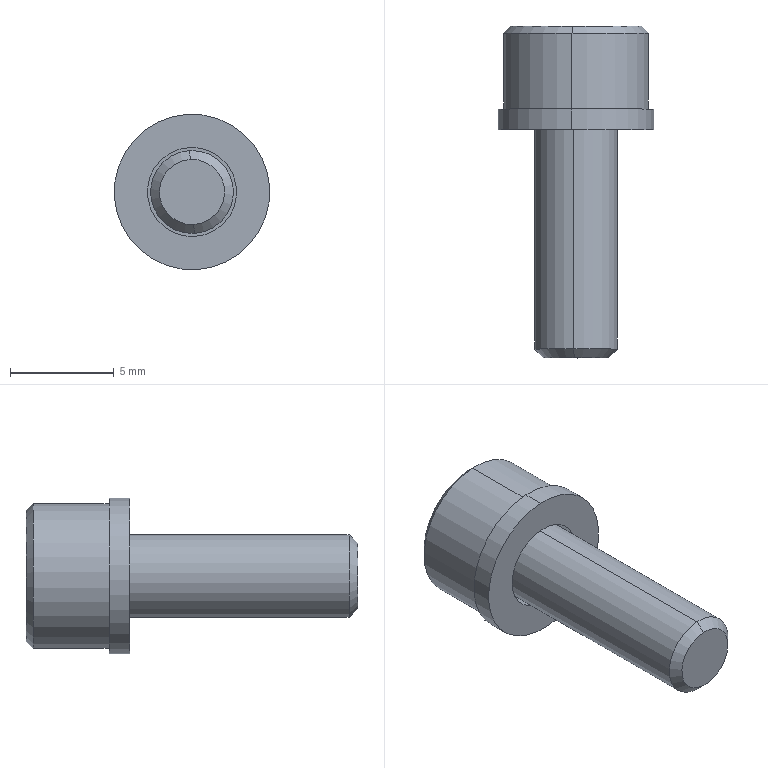Component | SolidWorks | TAC01-M4-L12-2 | 2 solids | 31 faces | box 7.5 x 16 x 7.5 mm | volume 314 mm3 | plane 17 | cylinder 8 | cone 6 | commonest cylinder face diameters 4.3 x2 7.5 x2 4 x2 7 x2
STEP:
#1=COLOUR_RGB('',0.7922,0.8196,0.9333);
#2=FILL_AREA_STYLE_COLOUR('',#1);
#3=FILL_AREA_STYLE('',(#2));
#4=SURFACE_STYLE_FILL_AREA(#3);
#5=SURFACE_SIDE_STYLE('',(#4));
#6=SURFACE_STYLE_USAGE(.BOTH.,#5);
#7=PRESENTATION_STYLE_ASSIGNMENT((#6));
#8=CARTESIAN_POINT('',(9.788,-21.078,0.1048));
#9=VERTEX_POINT('',#8);
#10=CARTESIAN_POINT('',(9.779,-21.078,0.2621));
#11=VERTEX_POINT('',#10);
#12=CARTESIAN_POINT('',(9.783,-21.078,0.1834));
#13=DIRECTION('',(0.,1.,-0.));
#14=DIRECTION('',(0.05512,0.,-0.9985));
#15=AXIS2_PLACEMENT_3D('',#12,#13,#14);
#16=CIRCLE('',#15,0.07874);
#17=EDGE_CURVE('',#9,#11,#16,.T.);
#18=ORIENTED_EDGE('',*,*,#17,.T.);
#19=CARTESIAN_POINT('',(9.779,-20.622,0.2621));
#20=VERTEX_POINT('',#19);
#21=CARTESIAN_POINT('',(9.779,-21.095,0.2621));
#22=DIRECTION('',(0.,1.,-0.));
#23=VECTOR('',#22,39.37);
#24=LINE('',#21,#23);
#25=EDGE_CURVE('',#11,#20,#24,.T.);
#26=ORIENTED_EDGE('',*,*,#25,.T.);
#27=CARTESIAN_POINT('',(9.788,-20.622,0.1048));
#28=VERTEX_POINT('',#27);
#29=CARTESIAN_POINT('',(9.783,-20.622,0.1834));
#30=DIRECTION('',(-0.,-1.,0.));
#31=DIRECTION('',(0.05512,0.,-0.9985));
#32=AXIS2_PLACEMENT_3D('',#29,#30,#31);
#33=CIRCLE('',#32,0.07874);
#34=EDGE_CURVE('',#20,#28,#33,.T.);
#35=ORIENTED_EDGE('',*,*,#34,.T.);
#36=CARTESIAN_POINT('',(9.788,-21.095,0.1048));
#37=DIRECTION('',(0.,1.,-0.));
#38=VECTOR('',#37,39.37);
#39=LINE('',#36,#38);
#40=EDGE_CURVE('',#9,#28,#39,.T.);
#41=ORIENTED_EDGE('',*,*,#40,.F.);
#42=EDGE_LOOP('',(#18,#26,#35,#41));
#43=FACE_OUTER_BOUND('',#42,.T.);
#44=CARTESIAN_POINT('',(9.783,-21.095,0.1834));
#45=DIRECTION('',(0.,1.,-0.));
#46=DIRECTION('',(0.05512,0.,-0.9985));
#47=AXIS2_PLACEMENT_3D('',#44,#45,#46);
#48=CYLINDRICAL_SURFACE('',#47,0.07874);
#49=ADVANCED_FACE('',(#43),#48,.T.);
#50=CARTESIAN_POINT('',(9.787,-21.095,0.1217));
#51=VERTEX_POINT('',#50);
#52=CARTESIAN_POINT('',(9.78,-21.095,0.2452));
#53=VERTEX_POINT('',#52);
#54=CARTESIAN_POINT('',(9.783,-21.095,0.1834));
#55=DIRECTION('',(0.,1.,-0.));
#56=DIRECTION('',(0.05512,0.,-0.9985));
#57=AXIS2_PLACEMENT_3D('',#54,#55,#56);
#58=CIRCLE('',#57,0.06183);
#59=EDGE_CURVE('',#51,#53,#58,.T.);
#60=ORIENTED_EDGE('',*,*,#59,.T.);
#61=CARTESIAN_POINT('',(9.779,-21.078,0.2621));
#62=DIRECTION('',(-0.03898,0.7071,0.706));
#63=VECTOR('',#62,39.37);
#64=LINE('',#61,#63);
#65=EDGE_CURVE('',#53,#11,#64,.T.);
#66=ORIENTED_EDGE('',*,*,#65,.T.);
#67=ORIENTED_EDGE('',*,*,#17,.F.);
#68=CARTESIAN_POINT('',(9.788,-21.078,0.1048));
#69=DIRECTION('',(0.03898,0.7071,-0.706));
#70=VECTOR('',#69,39.37);
#71=LINE('',#68,#70);
#72=EDGE_CURVE('',#51,#9,#71,.T.);
#73=ORIENTED_EDGE('',*,*,#72,.F.);
#74=EDGE_LOOP('',(#60,#66,#67,#73));
#75=FACE_OUTER_BOUND('',#74,.T.);
#76=CARTESIAN_POINT('',(9.783,-21.078,0.1834));
#77=DIRECTION('',(0.,1.,-0.));
#78=DIRECTION('',(0.05512,0.,-0.9985));
#79=AXIS2_PLACEMENT_3D('',#76,#77,#78);
#80=CONICAL_SURFACE('',#79,0.07874,0.7854);
#81=ADVANCED_FACE('',(#75),#80,.T.);
#82=CARTESIAN_POINT('',(9.791,-20.622,0.04586));
#83=VERTEX_POINT('',#82);
#84=CARTESIAN_POINT('',(9.776,-20.622,0.321));
#85=VERTEX_POINT('',#84);
#86=CARTESIAN_POINT('',(9.783,-20.622,0.1834));
#87=DIRECTION('',(0.,1.,-0.));
#88=DIRECTION('',(0.05512,0.,-0.9985));
#89=AXIS2_PLACEMENT_3D('',#86,#87,#88);
#90=CIRCLE('',#89,0.1378);
#91=EDGE_CURVE('',#83,#85,#90,.T.);
#92=ORIENTED_EDGE('',*,*,#91,.T.);
#93=CARTESIAN_POINT('',(9.776,-20.479,0.321));
#94=VERTEX_POINT('',#93);
#95=CARTESIAN_POINT('',(9.776,-20.622,0.321));
#96=DIRECTION('',(0.,1.,-0.));
#97=VECTOR('',#96,39.37);
#98=LINE('',#95,#97);
#99=EDGE_CURVE('',#85,#94,#98,.T.);
#100=ORIENTED_EDGE('',*,*,#99,.T.);
#101=CARTESIAN_POINT('',(9.791,-20.479,0.04586));
#102=VERTEX_POINT('',#101);
#103=CARTESIAN_POINT('',(9.783,-20.479,0.1834));
#104=DIRECTION('',(-0.,-1.,0.));
#105=DIRECTION('',(0.05512,0.,-0.9985));
#106=AXIS2_PLACEMENT_3D('',#103,#104,#105);
#107=CIRCLE('',#106,0.1378);
#108=EDGE_CURVE('',#94,#102,#107,.T.);
#109=ORIENTED_EDGE('',*,*,#108,.T.);
#110=CARTESIAN_POINT('',(9.791,-20.622,0.04586));
#111=DIRECTION('',(0.,1.,-0.));
#112=VECTOR('',#111,39.37);
#113=LINE('',#110,#112);
#114=EDGE_CURVE('',#83,#102,#113,.T.);
#115=ORIENTED_EDGE('',*,*,#114,.F.);
#116=EDGE_LOOP('',(#92,#100,#109,#115));
#117=FACE_OUTER_BOUND('',#116,.T.);
#118=CARTESIAN_POINT('',(9.783,-20.622,0.1834));
#119=DIRECTION('',(0.,1.,-0.));
#120=DIRECTION('',(0.05512,0.,-0.9985));
#121=AXIS2_PLACEMENT_3D('',#118,#119,#120);
#122=CYLINDRICAL_SURFACE('',#121,0.1378);
#123=ADVANCED_FACE('',(#117),#122,.T.);
#124=CARTESIAN_POINT('',(9.777,-20.465,0.3073));
#125=VERTEX_POINT('',#124);
#126=CARTESIAN_POINT('',(9.79,-20.465,0.05962));
#127=VERTEX_POINT('',#126);
#128=CARTESIAN_POINT('',(9.783,-20.465,0.1834));
#129=DIRECTION('',(-0.,-1.,0.));
#130=DIRECTION('',(-0.05512,0.,0.9985));
#131=AXIS2_PLACEMENT_3D('',#128,#129,#130);
#132=CIRCLE('',#131,0.124);
#133=EDGE_CURVE('',#125,#127,#132,.T.);
#134=ORIENTED_EDGE('',*,*,#133,.T.);
#135=CARTESIAN_POINT('',(9.791,-20.479,0.04586));
#136=DIRECTION('',(0.03898,-0.7071,-0.706));
#137=VECTOR('',#136,39.37);
#138=LINE('',#135,#137);
#139=EDGE_CURVE('',#127,#102,#138,.T.);
#140=ORIENTED_EDGE('',*,*,#139,.T.);
#141=ORIENTED_EDGE('',*,*,#108,.F.);
#142=CARTESIAN_POINT('',(9.776,-20.479,0.321));
#143=DIRECTION('',(-0.03898,-0.7071,0.706));
#144=VECTOR('',#143,39.37);
#145=LINE('',#142,#144);
#146=EDGE_CURVE('',#125,#94,#145,.T.);
#147=ORIENTED_EDGE('',*,*,#146,.F.);
#148=EDGE_LOOP('',(#134,#140,#141,#147));
#149=FACE_OUTER_BOUND('',#148,.T.);
#150=CARTESIAN_POINT('',(9.783,-20.479,0.1834));
#151=DIRECTION('',(-0.,-1.,0.));
#152=DIRECTION('',(-0.05512,0.,0.9985));
#153=AXIS2_PLACEMENT_3D('',#150,#151,#152);
#154=CONICAL_SURFACE('',#153,0.1378,0.7854);
#155=ADVANCED_FACE('',(#149),#154,.T.);
#156=CARTESIAN_POINT('',(9.783,-20.578,0.1834));
#157=VERTEX_POINT('',#156);
#158=CARTESIAN_POINT('',(9.842,-20.544,0.1867));
#159=VERTEX_POINT('',#158);
#160=CARTESIAN_POINT('',(9.842,-20.544,0.1867));
#161=DIRECTION('',(0.8647,0.5,0.04774));
#162=VECTOR('',#161,39.37);
#163=LINE('',#160,#162);
#164=EDGE_CURVE('',#157,#159,#163,.T.);
#165=ORIENTED_EDGE('',*,*,#164,.F.);
#166=CARTESIAN_POINT('',(9.724,-20.544,0.1802));
#167=VERTEX_POINT('',#166);
#168=CARTESIAN_POINT('',(9.724,-20.544,0.1802));
#169=DIRECTION('',(-0.8647,0.5,-0.04774));
#170=VECTOR('',#169,39.37);
#171=LINE('',#168,#170);
#172=EDGE_CURVE('',#157,#167,#171,.T.);
#173=ORIENTED_EDGE('',*,*,#172,.T.);
#174=CARTESIAN_POINT('',(9.731,-20.544,0.2101));
#175=VERTEX_POINT('',#174);
#176=CARTESIAN_POINT('',(9.783,-20.544,0.1834));
#177=DIRECTION('',(-0.,-1.,0.));
#178=DIRECTION('',(0.9985,0.,0.05512));
#179=AXIS2_PLACEMENT_3D('',#176,#177,#178);
#180=CIRCLE('',#179,0.05906);
#181=EDGE_CURVE('',#175,#167,#180,.T.);
#182=ORIENTED_EDGE('',*,*,#181,.F.);
#183=CARTESIAN_POINT('',(9.78,-20.544,0.2424));
#184=VERTEX_POINT('',#183);
#185=CARTESIAN_POINT('',(9.783,-20.544,0.1834));
#186=DIRECTION('',(-0.,-1.,0.));
#187=DIRECTION('',(0.9985,0.,0.05512));
#188=AXIS2_PLACEMENT_3D('',#185,#186,#187);
#189=CIRCLE('',#188,0.05906);
#190=EDGE_CURVE('',#184,#175,#189,.T.);
#191=ORIENTED_EDGE('',*,*,#190,.F.);
#192=CARTESIAN_POINT('',(9.833,-20.544,0.2157));
#193=VERTEX_POINT('',#192);
#194=CARTESIAN_POINT('',(9.783,-20.544,0.1834));
#195=DIRECTION('',(-0.,-1.,0.));
#196=DIRECTION('',(0.9985,0.,0.05512));
#197=AXIS2_PLACEMENT_3D('',#194,#195,#196);
#198=CIRCLE('',#197,0.05906);
#199=EDGE_CURVE('',#193,#184,#198,.T.);
#200=ORIENTED_EDGE('',*,*,#199,.F.);
#201=CARTESIAN_POINT('',(9.783,-20.544,0.1834));
#202=DIRECTION('',(-0.,-1.,0.));
#203=DIRECTION('',(0.9985,0.,0.05512));
#204=AXIS2_PLACEMENT_3D('',#201,#202,#203);
#205=CIRCLE('',#204,0.05906);
#206=EDGE_CURVE('',#159,#193,#205,.T.);
#207=ORIENTED_EDGE('',*,*,#206,.F.);
#208=EDGE_LOOP('',(#165,#173,#182,#191,#200,#207));
#209=FACE_OUTER_BOUND('',#208,.T.);
#210=CARTESIAN_POINT('',(9.783,-20.544,0.1834));
#211=DIRECTION('',(0.,1.,-0.));
#212=DIRECTION('',(0.9985,0.,0.05512));
#213=AXIS2_PLACEMENT_3D('',#210,#211,#212);
#214=CONICAL_SURFACE('',#213,0.05906,1.047);
#215=ADVANCED_FACE('',(#209),#214,.F.);
#216=ORIENTED_EDGE('',*,*,#25,.F.);
#217=CARTESIAN_POINT('',(9.783,-21.078,0.1834));
#218=DIRECTION('',(0.,1.,-0.));
#219=DIRECTION('',(0.05512,0.,-0.9985));
#220=AXIS2_PLACEMENT_3D('',#217,#218,#219);
#221=CIRCLE('',#220,0.07874);
#222=EDGE_CURVE('',#11,#9,#221,.T.);
#223=ORIENTED_EDGE('',*,*,#222,.T.);
#224=ORIENTED_EDGE('',*,*,#40,.T.);
#225=CARTESIAN_POINT('',(9.783,-20.622,0.1834));
#226=DIRECTION('',(-0.,-1.,0.));
#227=DIRECTION('',(0.05512,0.,-0.9985));
#228=AXIS2_PLACEMENT_3D('',#225,#226,#227);
#229=CIRCLE('',#228,0.07874);
#230=EDGE_CURVE('',#28,#20,#229,.T.);
#231=ORIENTED_EDGE('',*,*,#230,.T.);
#232=EDGE_LOOP('',(#216,#223,#224,#231));
#233=FACE_OUTER_BOUND('',#232,.T.);
#234=CARTESIAN_POINT('',(9.783,-21.095,0.1834));
#235=DIRECTION('',(0.,1.,-0.));
#236=DIRECTION('',(0.05512,0.,-0.9985));
#237=AXIS2_PLACEMENT_3D('',#234,#235,#236);
#238=CYLINDRICAL_SURFACE('',#237,0.07874);
#239=ADVANCED_FACE('',(#233),#238,.T.);
#240=ORIENTED_EDGE('',*,*,#91,.F.);
#241=CARTESIAN_POINT('',(9.783,-20.622,0.1834));
#242=DIRECTION('',(0.,1.,-0.));
#243=DIRECTION('',(0.05512,0.,-0.9985));
#244=AXIS2_PLACEMENT_3D('',#241,#242,#243);
#245=CIRCLE('',#244,0.1378);
#246=EDGE_CURVE('',#85,#83,#245,.T.);
#247=ORIENTED_EDGE('',*,*,#246,.F.);
#248=EDGE_LOOP('',(#240,#247));
#249=FACE_OUTER_BOUND('',#248,.T.);
#250=ORIENTED_EDGE('',*,*,#230,.F.);
#251=ORIENTED_EDGE('',*,*,#34,.F.);
#252=EDGE_LOOP('',(#250,#251));
#253=FACE_BOUND('',#252,.T.);
#254=CARTESIAN_POINT('',(9.646,-20.622,0.1759));
#255=DIRECTION('',(0.,1.,-0.));
#256=DIRECTION('',(0.05512,-0.,-0.9985));
#257=AXIS2_PLACEMENT_3D('',#254,#255,#256);
#258=PLANE('',#257);
#259=ADVANCED_FACE('',(#249,#253),#258,.F.);
#260=ORIENTED_EDGE('',*,*,#65,.F.);
#261=CARTESIAN_POINT('',(9.783,-21.095,0.1834));
#262=DIRECTION('',(0.,1.,-0.));
#263=DIRECTION('',(0.05512,0.,-0.9985));
#264=AXIS2_PLACEMENT_3D('',#261,#262,#263);
#265=CIRCLE('',#264,0.06183);
#266=EDGE_CURVE('',#53,#51,#265,.T.);
#267=ORIENTED_EDGE('',*,*,#266,.T.);
#268=ORIENTED_EDGE('',*,*,#72,.T.);
#269=ORIENTED_EDGE('',*,*,#222,.F.);
#270=EDGE_LOOP('',(#260,#267,#268,#269));
#271=FACE_OUTER_BOUND('',#270,.T.);
#272=CARTESIAN_POINT('',(9.783,-21.078,0.1834));
#273=DIRECTION('',(0.,1.,-0.));
#274=DIRECTION('',(0.05512,0.,-0.9985));
#275=AXIS2_PLACEMENT_3D('',#272,#273,#274);
#276=CONICAL_SURFACE('',#275,0.07874,0.7854);
#277=ADVANCED_FACE('',(#271),#276,.T.);
#278=ORIENTED_EDGE('',*,*,#99,.F.);
#279=ORIENTED_EDGE('',*,*,#246,.T.);
#280=ORIENTED_EDGE('',*,*,#114,.T.);
#281=CARTESIAN_POINT('',(9.783,-20.479,0.1834));
#282=DIRECTION('',(-0.,-1.,0.));
#283=DIRECTION('',(0.05512,0.,-0.9985));
#284=AXIS2_PLACEMENT_3D('',#281,#282,#283);
#285=CIRCLE('',#284,0.1378);
#286=EDGE_CURVE('',#102,#94,#285,.T.);
#287=ORIENTED_EDGE('',*,*,#286,.T.);
#288=EDGE_LOOP('',(#278,#279,#280,#287));
#289=FACE_OUTER_BOUND('',#288,.T.);
#290=CARTESIAN_POINT('',(9.783,-20.622,0.1834));
#291=DIRECTION('',(0.,1.,-0.));
#292=DIRECTION('',(0.05512,0.,-0.9985));
#293=AXIS2_PLACEMENT_3D('',#290,#291,#292);
#294=CYLINDRICAL_SURFACE('',#293,0.1378);
#295=ADVANCED_FACE('',(#289),#294,.T.);
#296=ORIENTED_EDGE('',*,*,#59,.F.);
#297=ORIENTED_EDGE('',*,*,#266,.F.);
#298=EDGE_LOOP('',(#296,#297));
#299=FACE_OUTER_BOUND('',#298,.T.);
#300=CARTESIAN_POINT('',(9.722,-21.095,0.18));
#301=DIRECTION('',(0.,1.,-0.));
#302=DIRECTION('',(0.05512,-0.,-0.9985));
#303=AXIS2_PLACEMENT_3D('',#300,#301,#302);
#304=PLANE('',#303);
#305=ADVANCED_FACE('',(#299),#304,.F.);
#306=ORIENTED_EDGE('',*,*,#139,.F.);
#307=CARTESIAN_POINT('',(9.783,-20.465,0.1834));
#308=DIRECTION('',(-0.,-1.,0.));
#309=DIRECTION('',(-0.05512,0.,0.9985));
#310=AXIS2_PLACEMENT_3D('',#307,#308,#309);
#311=CIRCLE('',#310,0.124);
#312=EDGE_CURVE('',#127,#125,#311,.T.);
#313=ORIENTED_EDGE('',*,*,#312,.T.);
#314=ORIENTED_EDGE('',*,*,#146,.T.);
#315=ORIENTED_EDGE('',*,*,#286,.F.);
#316=EDGE_LOOP('',(#306,#313,#314,#315));
#317=FACE_OUTER_BOUND('',#316,.T.);
#318=CARTESIAN_POINT('',(9.783,-20.479,0.1834));
#319=DIRECTION('',(-0.,-1.,0.));
#320=DIRECTION('',(-0.05512,0.,0.9985));
#321=AXIS2_PLACEMENT_3D('',#318,#319,#320);
#322=CONICAL_SURFACE('',#321,0.1378,0.7854);
#323=ADVANCED_FACE('',(#317),#322,.T.);
#324=CARTESIAN_POINT('',(9.852,-20.465,0.1872));
#325=VERTEX_POINT('',#324);
#326=CARTESIAN_POINT('',(9.814,-20.465,0.2443));
#327=VERTEX_POINT('',#326);
#328=CARTESIAN_POINT('',(9.814,-20.465,0.2443));
#329=DIRECTION('',(-0.547,0.,0.8371));
#330=VECTOR('',#329,39.37);
#331=LINE('',#328,#330);
#332=EDGE_CURVE('',#325,#327,#331,.T.);
#333=ORIENTED_EDGE('',*,*,#332,.T.);
#334=CARTESIAN_POINT('',(9.746,-20.465,0.2405));
#335=VERTEX_POINT('',#334);
#336=CARTESIAN_POINT('',(9.746,-20.465,0.2405));
#337=DIRECTION('',(-0.9985,0.,-0.05512));
#338=VECTOR('',#337,39.37);
#339=LINE('',#336,#338);
#340=EDGE_CURVE('',#327,#335,#339,.T.);
#341=ORIENTED_EDGE('',*,*,#340,.T.);
#342=CARTESIAN_POINT('',(9.715,-20.465,0.1797));
#343=VERTEX_POINT('',#342);
#344=CARTESIAN_POINT('',(9.715,-20.465,0.1797));
#345=DIRECTION('',(-0.4515,0.,-0.8923));
#346=VECTOR('',#345,39.37);
#347=LINE('',#344,#346);
#348=EDGE_CURVE('',#335,#343,#347,.T.);
#349=ORIENTED_EDGE('',*,*,#348,.T.);
#350=CARTESIAN_POINT('',(9.753,-20.465,0.1226));
#351=VERTEX_POINT('',#350);
#352=CARTESIAN_POINT('',(9.753,-20.465,0.1226));
#353=DIRECTION('',(0.547,-0.,-0.8371));
#354=VECTOR('',#353,39.37);
#355=LINE('',#352,#354);
#356=EDGE_CURVE('',#343,#351,#355,.T.);
#357=ORIENTED_EDGE('',*,*,#356,.T.);
#358=CARTESIAN_POINT('',(9.821,-20.465,0.1264));
#359=VERTEX_POINT('',#358);
#360=CARTESIAN_POINT('',(9.821,-20.465,0.1264));
#361=DIRECTION('',(0.9985,-0.,0.05512));
#362=VECTOR('',#361,39.37);
#363=LINE('',#360,#362);
#364=EDGE_CURVE('',#351,#359,#363,.T.);
#365=ORIENTED_EDGE('',*,*,#364,.T.);
#366=CARTESIAN_POINT('',(9.852,-20.465,0.1872));
#367=DIRECTION('',(-0.4515,0.,-0.8923));
#368=VECTOR('',#367,39.37);
#369=LINE('',#366,#368);
#370=EDGE_CURVE('',#325,#359,#369,.T.);
#371=ORIENTED_EDGE('',*,*,#370,.F.);
#372=EDGE_LOOP('',(#333,#341,#349,#357,#365,#371));
#373=FACE_BOUND('',#372,.T.);
#374=ORIENTED_EDGE('',*,*,#133,.F.);
#375=ORIENTED_EDGE('',*,*,#312,.F.);
#376=EDGE_LOOP('',(#374,#375));
#377=FACE_OUTER_BOUND('',#376,.T.);
#378=CARTESIAN_POINT('',(9.783,-20.465,0.1834));
#379=DIRECTION('',(-0.,-1.,0.));
#380=DIRECTION('',(-0.05512,0.,0.9985));
#381=AXIS2_PLACEMENT_3D('',#378,#379,#380);
#382=PLANE('',#381);
#383=ADVANCED_FACE('',(#373,#377),#382,.F.);
#384=CARTESIAN_POINT('',(9.821,-20.544,0.1264));
#385=VERTEX_POINT('',#384);
#386=CARTESIAN_POINT('',(9.821,-20.544,0.1264));
#387=DIRECTION('',(0.,1.,-0.));
#388=VECTOR('',#387,39.37);
#389=LINE('',#386,#388);
#390=EDGE_CURVE('',#385,#359,#389,.T.);
#391=ORIENTED_EDGE('',*,*,#390,.F.);
#392=CARTESIAN_POINT('',(9.836,-20.544,0.1568));
#393=VERTEX_POINT('',#392);
#394=CARTESIAN_POINT('',(9.852,-20.544,0.1872));
#395=DIRECTION('',(-0.4515,0.,-0.8923));
#396=VECTOR('',#395,39.37);
#397=LINE('',#394,#396);
#398=EDGE_CURVE('',#393,#385,#397,.T.);
#399=ORIENTED_EDGE('',*,*,#398,.F.);
#400=CARTESIAN_POINT('',(9.852,-20.544,0.1872));
#401=VERTEX_POINT('',#400);
#402=CARTESIAN_POINT('',(9.852,-20.544,0.1872));
#403=DIRECTION('',(-0.4515,0.,-0.8923));
#404=VECTOR('',#403,39.37);
#405=LINE('',#402,#404);
#406=EDGE_CURVE('',#401,#393,#405,.T.);
#407=ORIENTED_EDGE('',*,*,#406,.F.);
#408=CARTESIAN_POINT('',(9.852,-20.544,0.1872));
#409=DIRECTION('',(-0.,-1.,0.));
#410=VECTOR('',#409,39.37);
#411=LINE('',#408,#410);
#412=EDGE_CURVE('',#325,#401,#411,.T.);
#413=ORIENTED_EDGE('',*,*,#412,.F.);
#414=ORIENTED_EDGE('',*,*,#370,.T.);
#415=EDGE_LOOP('',(#391,#399,#407,#413,#414));
#416=FACE_OUTER_BOUND('',#415,.T.);
#417=CARTESIAN_POINT('',(9.852,-20.544,0.1872));
#418=DIRECTION('',(0.8923,-0.,-0.4515));
#419=DIRECTION('',(-0.4515,0.,-0.8923));
#420=AXIS2_PLACEMENT_3D('',#417,#418,#419);
#421=PLANE('',#420);
#422=ADVANCED_FACE('',(#416),#421,.F.);
#423=CARTESIAN_POINT('',(9.753,-20.544,0.1226));
#424=VERTEX_POINT('',#423);
#425=CARTESIAN_POINT('',(9.753,-20.544,0.1226));
#426=DIRECTION('',(0.,1.,-0.));
#427=VECTOR('',#426,39.37);
#428=LINE('',#425,#427);
#429=EDGE_CURVE('',#424,#351,#428,.T.);
#430=ORIENTED_EDGE('',*,*,#429,.F.);
#431=CARTESIAN_POINT('',(9.787,-20.544,0.1245));
#432=VERTEX_POINT('',#431);
#433=CARTESIAN_POINT('',(9.821,-20.544,0.1264));
#434=DIRECTION('',(-0.9985,0.,-0.05512));
#435=VECTOR('',#434,39.37);
#436=LINE('',#433,#435);
#437=EDGE_CURVE('',#432,#424,#436,.T.);
#438=ORIENTED_EDGE('',*,*,#437,.F.);
#439=CARTESIAN_POINT('',(9.821,-20.544,0.1264));
#440=DIRECTION('',(-0.9985,0.,-0.05512));
#441=VECTOR('',#440,39.37);
#442=LINE('',#439,#441);
#443=EDGE_CURVE('',#385,#432,#442,.T.);
#444=ORIENTED_EDGE('',*,*,#443,.F.);
#445=ORIENTED_EDGE('',*,*,#390,.T.);
#446=ORIENTED_EDGE('',*,*,#364,.F.);
#447=EDGE_LOOP('',(#430,#438,#444,#445,#446));
#448=FACE_OUTER_BOUND('',#447,.T.);
#449=CARTESIAN_POINT('',(9.821,-20.544,0.1264));
#450=DIRECTION('',(0.05512,-0.,-0.9985));
#451=DIRECTION('',(-0.,-1.,0.));
#452=AXIS2_PLACEMENT_3D('',#449,#450,#451);
#453=PLANE('',#452);
#454=ADVANCED_FACE('',(#448),#453,.F.);
#455=CARTESIAN_POINT('',(9.783,-20.544,0.1834));
#456=DIRECTION('',(-0.,-1.,0.));
#457=DIRECTION('',(0.9985,0.,0.05512));
#458=AXIS2_PLACEMENT_3D('',#455,#456,#457);
#459=CIRCLE('',#458,0.05906);
#460=EDGE_CURVE('',#432,#393,#459,.T.);
#461=ORIENTED_EDGE('',*,*,#460,.T.);
#462=ORIENTED_EDGE('',*,*,#398,.T.);
#463=ORIENTED_EDGE('',*,*,#443,.T.);
#464=EDGE_LOOP('',(#461,#462,#463));
#465=FACE_OUTER_BOUND('',#464,.T.);
#466=CARTESIAN_POINT('',(9.783,-20.544,0.1834));
#467=DIRECTION('',(0.,1.,-0.));
#468=DIRECTION('',(0.05512,-0.,-0.9985));
#469=AXIS2_PLACEMENT_3D('',#466,#467,#468);
#470=PLANE('',#469);
#471=ADVANCED_FACE('',(#465),#470,.T.);
#472=CARTESIAN_POINT('',(9.783,-20.544,0.1834));
#473=DIRECTION('',(-0.,-1.,0.));
#474=DIRECTION('',(0.9985,0.,0.05512));
#475=AXIS2_PLACEMENT_3D('',#472,#473,#474);
#476=CIRCLE('',#475,0.05906);
#477=EDGE_CURVE('',#393,#159,#476,.T.);
#478=ORIENTED_EDGE('',*,*,#477,.T.);
#479=ORIENTED_EDGE('',*,*,#206,.T.);
#480=CARTESIAN_POINT('',(9.833,-20.544,0.2157));
#481=DIRECTION('',(0.547,-0.,-0.8371));
#482=VECTOR('',#481,39.37);
#483=LINE('',#480,#482);
#484=EDGE_CURVE('',#193,#401,#483,.T.);
#485=ORIENTED_EDGE('',*,*,#484,.T.);
#486=ORIENTED_EDGE('',*,*,#406,.T.);
#487=EDGE_LOOP('',(#478,#479,#485,#486));
#488=FACE_OUTER_BOUND('',#487,.T.);
#489=CARTESIAN_POINT('',(9.783,-20.544,0.1834));
#490=DIRECTION('',(0.,1.,-0.));
#491=DIRECTION('',(0.05512,-0.,-0.9985));
#492=AXIS2_PLACEMENT_3D('',#489,#490,#491);
#493=PLANE('',#492);
#494=ADVANCED_FACE('',(#488),#493,.T.);
#495=ORIENTED_EDGE('',*,*,#412,.T.);
#496=ORIENTED_EDGE('',*,*,#484,.F.);
#497=CARTESIAN_POINT('',(9.814,-20.544,0.2443));
#498=VERTEX_POINT('',#497);
#499=CARTESIAN_POINT('',(9.814,-20.544,0.2443));
#500=DIRECTION('',(0.547,-0.,-0.8371));
#501=VECTOR('',#500,39.37);
#502=LINE('',#499,#501);
#503=EDGE_CURVE('',#498,#193,#502,.T.);
#504=ORIENTED_EDGE('',*,*,#503,.F.);
#505=CARTESIAN_POINT('',(9.814,-20.544,0.2443));
#506=DIRECTION('',(-0.,-1.,0.));
#507=VECTOR('',#506,39.37);
#508=LINE('',#505,#507);
#509=EDGE_CURVE('',#327,#498,#508,.T.);
#510=ORIENTED_EDGE('',*,*,#509,.F.);
#511=ORIENTED_EDGE('',*,*,#332,.F.);
#512=EDGE_LOOP('',(#495,#496,#504,#510,#511));
#513=FACE_OUTER_BOUND('',#512,.T.);
#514=CARTESIAN_POINT('',(9.814,-20.544,0.2443));
#515=DIRECTION('',(0.8371,-0.,0.547));
#516=DIRECTION('',(0.547,-0.,-0.8371));
#517=AXIS2_PLACEMENT_3D('',#514,#515,#516);
#518=PLANE('',#517);
#519=ADVANCED_FACE('',(#513),#518,.F.);
#520=CARTESIAN_POINT('',(9.715,-20.544,0.1797));
#521=VERTEX_POINT('',#520);
#522=CARTESIAN_POINT('',(9.715,-20.544,0.1797));
#523=DIRECTION('',(0.,1.,-0.));
#524=VECTOR('',#523,39.37);
#525=LINE('',#522,#524);
#526=EDGE_CURVE('',#521,#343,#525,.T.);
#527=ORIENTED_EDGE('',*,*,#526,.F.);
#528=CARTESIAN_POINT('',(9.734,-20.544,0.1511));
#529=VERTEX_POINT('',#528);
#530=CARTESIAN_POINT('',(9.753,-20.544,0.1226));
#531=DIRECTION('',(-0.547,0.,0.8371));
#532=VECTOR('',#531,39.37);
#533=LINE('',#530,#532);
#534=EDGE_CURVE('',#529,#521,#533,.T.);
#535=ORIENTED_EDGE('',*,*,#534,.F.);
#536=CARTESIAN_POINT('',(9.753,-20.544,0.1226));
#537=DIRECTION('',(-0.547,0.,0.8371));
#538=VECTOR('',#537,39.37);
#539=LINE('',#536,#538);
#540=EDGE_CURVE('',#424,#529,#539,.T.);
#541=ORIENTED_EDGE('',*,*,#540,.F.);
#542=ORIENTED_EDGE('',*,*,#429,.T.);
#543=ORIENTED_EDGE('',*,*,#356,.F.);
#544=EDGE_LOOP('',(#527,#535,#541,#542,#543));
#545=FACE_OUTER_BOUND('',#544,.T.);
#546=CARTESIAN_POINT('',(9.753,-20.544,0.1226));
#547=DIRECTION('',(-0.8371,0.,-0.547));
#548=DIRECTION('',(-0.547,0.,0.8371));
#549=AXIS2_PLACEMENT_3D('',#546,#547,#548);
#550=PLANE('',#549);
#551=ADVANCED_FACE('',(#545),#550,.F.);
#552=CARTESIAN_POINT('',(9.783,-20.544,0.1834));
#553=DIRECTION('',(-0.,-1.,0.));
#554=DIRECTION('',(0.9985,0.,0.05512));
#555=AXIS2_PLACEMENT_3D('',#552,#553,#554);
#556=CIRCLE('',#555,0.05906);
#557=EDGE_CURVE('',#529,#432,#556,.T.);
#558=ORIENTED_EDGE('',*,*,#557,.T.);
#559=ORIENTED_EDGE('',*,*,#437,.T.);
#560=ORIENTED_EDGE('',*,*,#540,.T.);
#561=EDGE_LOOP('',(#558,#559,#560));
#562=FACE_OUTER_BOUND('',#561,.T.);
#563=CARTESIAN_POINT('',(9.783,-20.544,0.1834));
#564=DIRECTION('',(0.,1.,-0.));
#565=DIRECTION('',(0.05512,-0.,-0.9985));
#566=AXIS2_PLACEMENT_3D('',#563,#564,#565);
#567=PLANE('',#566);
#568=ADVANCED_FACE('',(#562),#567,.T.);
#569=ORIENTED_EDGE('',*,*,#172,.F.);
#570=ORIENTED_EDGE('',*,*,#164,.T.);
#571=ORIENTED_EDGE('',*,*,#477,.F.);
#572=ORIENTED_EDGE('',*,*,#460,.F.);
#573=ORIENTED_EDGE('',*,*,#557,.F.);
#574=CARTESIAN_POINT('',(9.783,-20.544,0.1834));
#575=DIRECTION('',(-0.,-1.,0.));
#576=DIRECTION('',(0.9985,0.,0.05512));
#577=AXIS2_PLACEMENT_3D('',#574,#575,#576);
#578=CIRCLE('',#577,0.05906);
#579=EDGE_CURVE('',#167,#529,#578,.T.);
#580=ORIENTED_EDGE('',*,*,#579,.F.);
#581=EDGE_LOOP('',(#569,#570,#571,#572,#573,#580));
#582=FACE_OUTER_BOUND('',#581,.T.);
#583=CARTESIAN_POINT('',(9.783,-20.544,0.1834));
#584=DIRECTION('',(0.,1.,-0.));
#585=DIRECTION('',(0.9985,0.,0.05512));
#586=AXIS2_PLACEMENT_3D('',#583,#584,#585);
#587=CONICAL_SURFACE('',#586,0.05906,1.047);
#588=ADVANCED_FACE('',(#582),#587,.F.);
#589=ORIENTED_EDGE('',*,*,#199,.T.);
#590=CARTESIAN_POINT('',(9.78,-20.544,0.2424));
#591=DIRECTION('',(0.9985,-0.,0.05512));
#592=VECTOR('',#591,39.37);
#593=LINE('',#590,#592);
#594=EDGE_CURVE('',#184,#498,#593,.T.);
#595=ORIENTED_EDGE('',*,*,#594,.T.);
#596=ORIENTED_EDGE('',*,*,#503,.T.);
#597=EDGE_LOOP('',(#589,#595,#596));
#598=FACE_OUTER_BOUND('',#597,.T.);
#599=CARTESIAN_POINT('',(9.783,-20.544,0.1834));
#600=DIRECTION('',(0.,1.,-0.));
#601=DIRECTION('',(0.05512,-0.,-0.9985));
#602=AXIS2_PLACEMENT_3D('',#599,#600,#601);
#603=PLANE('',#602);
#604=ADVANCED_FACE('',(#598),#603,.T.);
#605=ORIENTED_EDGE('',*,*,#509,.T.);
#606=ORIENTED_EDGE('',*,*,#594,.F.);
#607=CARTESIAN_POINT('',(9.746,-20.544,0.2405));
#608=VERTEX_POINT('',#607);
#609=CARTESIAN_POINT('',(9.746,-20.544,0.2405));
#610=DIRECTION('',(0.9985,-0.,0.05512));
#611=VECTOR('',#610,39.37);
#612=LINE('',#609,#611);
#613=EDGE_CURVE('',#608,#184,#612,.T.);
#614=ORIENTED_EDGE('',*,*,#613,.F.);
#615=CARTESIAN_POINT('',(9.746,-20.544,0.2405));
#616=DIRECTION('',(-0.,-1.,0.));
#617=VECTOR('',#616,39.37);
#618=LINE('',#615,#617);
#619=EDGE_CURVE('',#335,#608,#618,.T.);
#620=ORIENTED_EDGE('',*,*,#619,.F.);
#621=ORIENTED_EDGE('',*,*,#340,.F.);
#622=EDGE_LOOP('',(#605,#606,#614,#620,#621));
#623=FACE_OUTER_BOUND('',#622,.T.);
#624=CARTESIAN_POINT('',(9.746,-20.544,0.2405));
#625=DIRECTION('',(-0.05512,0.,0.9985));
#626=DIRECTION('',(0.,1.,-0.));
#627=AXIS2_PLACEMENT_3D('',#624,#625,#626);
#628=PLANE('',#627);
#629=ADVANCED_FACE('',(#623),#628,.F.);
#630=ORIENTED_EDGE('',*,*,#619,.T.);
#631=CARTESIAN_POINT('',(9.715,-20.544,0.1797));
#632=DIRECTION('',(0.4515,-0.,0.8923));
#633=VECTOR('',#632,39.37);
#634=LINE('',#631,#633);
#635=EDGE_CURVE('',#175,#608,#634,.T.);
#636=ORIENTED_EDGE('',*,*,#635,.F.);
#637=CARTESIAN_POINT('',(9.715,-20.544,0.1797));
#638=DIRECTION('',(0.4515,-0.,0.8923));
#639=VECTOR('',#638,39.37);
#640=LINE('',#637,#639);
#641=EDGE_CURVE('',#521,#175,#640,.T.);
#642=ORIENTED_EDGE('',*,*,#641,.F.);
#643=ORIENTED_EDGE('',*,*,#526,.T.);
#644=ORIENTED_EDGE('',*,*,#348,.F.);
#645=EDGE_LOOP('',(#630,#636,#642,#643,#644));
#646=FACE_OUTER_BOUND('',#645,.T.);
#647=CARTESIAN_POINT('',(9.715,-20.544,0.1797));
#648=DIRECTION('',(-0.8923,0.,0.4515));
#649=DIRECTION('',(0.4515,-0.,0.8923));
#650=AXIS2_PLACEMENT_3D('',#647,#648,#649);
#651=PLANE('',#650);
#652=ADVANCED_FACE('',(#646),#651,.F.);
#653=ORIENTED_EDGE('',*,*,#181,.T.);
#654=ORIENTED_EDGE('',*,*,#579,.T.);
#655=ORIENTED_EDGE('',*,*,#534,.T.);
#656=ORIENTED_EDGE('',*,*,#641,.T.);
#657=EDGE_LOOP('',(#653,#654,#655,#656));
#658=FACE_OUTER_BOUND('',#657,.T.);
#659=CARTESIAN_POINT('',(9.783,-20.544,0.1834));
#660=DIRECTION('',(0.,1.,-0.));
#661=DIRECTION('',(0.05512,-0.,-0.9985));
#662=AXIS2_PLACEMENT_3D('',#659,#660,#661);
#663=PLANE('',#662);
#664=ADVANCED_FACE('',(#658),#663,.T.);
#665=ORIENTED_EDGE('',*,*,#190,.T.);
#666=ORIENTED_EDGE('',*,*,#635,.T.);
#667=ORIENTED_EDGE('',*,*,#613,.T.);
#668=EDGE_LOOP('',(#665,#666,#667));
#669=FACE_OUTER_BOUND('',#668,.T.);
#670=CARTESIAN_POINT('',(9.783,-20.544,0.1834));
#671=DIRECTION('',(0.,1.,-0.));
#672=DIRECTION('',(0.05512,-0.,-0.9985));
#673=AXIS2_PLACEMENT_3D('',#670,#671,#672);
#674=PLANE('',#673);
#675=ADVANCED_FACE('',(#669),#674,.T.);
#676=CLOSED_SHELL('',(#49,#81,#123,#155,#215,#239,#259,#277,#295,#305,#323,#383,#422,#454,#471,#494,#519,#551,#568,#588,#604,#629,#652,#664,#675));
#677=MANIFOLD_SOLID_BREP('',#676);
#678=STYLED_ITEM('',(#7),#677);
#679=PRESENTATION_LAYER_ASSIGNMENT('','',(#678));
#680=(LENGTH_UNIT()NAMED_UNIT(*)SI_UNIT($,.METRE.));
#681=LENGTH_MEASURE_WITH_UNIT(LENGTH_MEASURE(0.0254),#680);
#682=DIMENSIONAL_EXPONENTS(1.,0.,0.,0.,0.,0.,0.);
#683=(CONVERSION_BASED_UNIT('',#681)LENGTH_UNIT()NAMED_UNIT(#682));
#684=UNCERTAINTY_MEASURE_WITH_UNIT(LENGTH_MEASURE(0.00001),#683,'','');
#685=(NAMED_UNIT(*)PLANE_ANGLE_UNIT()SI_UNIT($,.RADIAN.));
#686=(NAMED_UNIT(*)SI_UNIT($,.STERADIAN.)SOLID_ANGLE_UNIT());
#687=(GEOMETRIC_REPRESENTATION_CONTEXT(3)GLOBAL_UNCERTAINTY_ASSIGNED_CONTEXT((#684))GLOBAL_UNIT_ASSIGNED_CONTEXT((#683,#685,#686))REPRESENTATION_CONTEXT('',''));
#688=MECHANICAL_DESIGN_GEOMETRIC_PRESENTATION_REPRESENTATION('',(#678),#687);
#689=COLOUR_RGB('',0.7922,0.8196,0.9333);
#690=FILL_AREA_STYLE_COLOUR('',#689);
#691=FILL_AREA_STYLE('',(#690));
#692=SURFACE_STYLE_FILL_AREA(#691);
#693=SURFACE_SIDE_STYLE('',(#692));
#694=SURFACE_STYLE_USAGE(.BOTH.,#693);
#695=PRESENTATION_STYLE_ASSIGNMENT((#694));
#696=CARTESIAN_POINT('',(9.788,-20.662,0.09893));
#697=VERTEX_POINT('',#696);
#698=CARTESIAN_POINT('',(9.779,-20.662,0.268));
#699=VERTEX_POINT('',#698);
#700=CARTESIAN_POINT('',(9.783,-20.662,0.1834));
#701=DIRECTION('',(-0.,-1.,0.));
#702=DIRECTION('',(-0.05512,0.,0.9985));
#703=AXIS2_PLACEMENT_3D('',#700,#701,#702);
#704=CIRCLE('',#703,0.08465);
#705=EDGE_CURVE('',#697,#699,#704,.T.);
#706=ORIENTED_EDGE('',*,*,#705,.T.);
#707=CARTESIAN_POINT('',(9.779,-20.622,0.268));
#708=VERTEX_POINT('',#707);
#709=CARTESIAN_POINT('',(9.779,-20.662,0.268));
#710=DIRECTION('',(0.,1.,-0.));
#711=VECTOR('',#710,39.37);
#712=LINE('',#709,#711);
#713=EDGE_CURVE('',#699,#708,#712,.T.);
#714=ORIENTED_EDGE('',*,*,#713,.T.);
#715=CARTESIAN_POINT('',(9.788,-20.622,0.09893));
#716=VERTEX_POINT('',#715);
#717=CARTESIAN_POINT('',(9.783,-20.622,0.1834));
#718=DIRECTION('',(-0.,-1.,0.));
#719=DIRECTION('',(-0.05512,0.,0.9985));
#720=AXIS2_PLACEMENT_3D('',#717,#718,#719);
#721=CIRCLE('',#720,0.08465);
#722=EDGE_CURVE('',#716,#708,#721,.T.);
#723=ORIENTED_EDGE('',*,*,#722,.F.);
#724=CARTESIAN_POINT('',(9.788,-20.662,0.09893));
#725=DIRECTION('',(0.,1.,-0.));
#726=VECTOR('',#725,39.37);
#727=LINE('',#724,#726);
#728=EDGE_CURVE('',#697,#716,#727,.T.);
#729=ORIENTED_EDGE('',*,*,#728,.F.);
#730=EDGE_LOOP('',(#706,#714,#723,#729));
#731=FACE_OUTER_BOUND('',#730,.T.);
#732=CARTESIAN_POINT('',(9.783,-20.662,0.1834));
#733=DIRECTION('',(0.,1.,-0.));
#734=DIRECTION('',(0.05512,0.,-0.9985));
#735=AXIS2_PLACEMENT_3D('',#732,#733,#734);
#736=CYLINDRICAL_SURFACE('',#735,0.08465);
#737=ADVANCED_FACE('',(#731),#736,.F.);
#738=CARTESIAN_POINT('',(9.775,-20.662,0.3309));
#739=VERTEX_POINT('',#738);
#740=CARTESIAN_POINT('',(9.792,-20.662,0.03603));
#741=VERTEX_POINT('',#740);
#742=CARTESIAN_POINT('',(9.783,-20.662,0.1834));
#743=DIRECTION('',(-0.,-1.,0.));
#744=DIRECTION('',(-0.05512,0.,0.9985));
#745=AXIS2_PLACEMENT_3D('',#742,#743,#744);
#746=CIRCLE('',#745,0.1476);
#747=EDGE_CURVE('',#739,#741,#746,.T.);
#748=ORIENTED_EDGE('',*,*,#747,.F.);
#749=CARTESIAN_POINT('',(9.775,-20.622,0.3309));
#750=VERTEX_POINT('',#749);
#751=CARTESIAN_POINT('',(9.775,-20.662,0.3309));
#752=DIRECTION('',(0.,1.,-0.));
#753=VECTOR('',#752,39.37);
#754=LINE('',#751,#753);
#755=EDGE_CURVE('',#739,#750,#754,.T.);
#756=ORIENTED_EDGE('',*,*,#755,.T.);
#757=CARTESIAN_POINT('',(9.792,-20.622,0.03603));
#758=VERTEX_POINT('',#757);
#759=CARTESIAN_POINT('',(9.783,-20.622,0.1834));
#760=DIRECTION('',(-0.,-1.,0.));
#761=DIRECTION('',(-0.05512,0.,0.9985));
#762=AXIS2_PLACEMENT_3D('',#759,#760,#761);
#763=CIRCLE('',#762,0.1476);
#764=EDGE_CURVE('',#750,#758,#763,.T.);
#765=ORIENTED_EDGE('',*,*,#764,.T.);
#766=CARTESIAN_POINT('',(9.792,-20.662,0.03603));
#767=DIRECTION('',(0.,1.,-0.));
#768=VECTOR('',#767,39.37);
#769=LINE('',#766,#768);
#770=EDGE_CURVE('',#741,#758,#769,.T.);
#771=ORIENTED_EDGE('',*,*,#770,.F.);
#772=EDGE_LOOP('',(#748,#756,#765,#771));
#773=FACE_OUTER_BOUND('',#772,.T.);
#774=CARTESIAN_POINT('',(9.783,-20.662,0.1834));
#775=DIRECTION('',(0.,1.,-0.));
#776=DIRECTION('',(0.05512,0.,-0.9985));
#777=AXIS2_PLACEMENT_3D('',#774,#775,#776);
#778=CYLINDRICAL_SURFACE('',#777,0.1476);
#779=ADVANCED_FACE('',(#773),#778,.T.);
#780=CARTESIAN_POINT('',(9.783,-20.662,0.1834));
#781=DIRECTION('',(-0.,-1.,0.));
#782=DIRECTION('',(-0.05512,0.,0.9985));
#783=AXIS2_PLACEMENT_3D('',#780,#781,#782);
#784=CIRCLE('',#783,0.1476);
#785=EDGE_CURVE('',#741,#739,#784,.T.);
#786=ORIENTED_EDGE('',*,*,#785,.T.);
#787=ORIENTED_EDGE('',*,*,#747,.T.);
#788=EDGE_LOOP('',(#786,#787));
#789=FACE_OUTER_BOUND('',#788,.T.);
#790=ORIENTED_EDGE('',*,*,#705,.F.);
#791=CARTESIAN_POINT('',(9.783,-20.662,0.1834));
#792=DIRECTION('',(-0.,-1.,0.));
#793=DIRECTION('',(-0.05512,0.,0.9985));
#794=AXIS2_PLACEMENT_3D('',#791,#792,#793);
#795=CIRCLE('',#794,0.08465);
#796=EDGE_CURVE('',#699,#697,#795,.T.);
#797=ORIENTED_EDGE('',*,*,#796,.F.);
#798=EDGE_LOOP('',(#790,#797));
#799=FACE_BOUND('',#798,.T.);
#800=CARTESIAN_POINT('',(9.783,-20.662,0.1834));
#801=DIRECTION('',(-0.,-1.,0.));
#802=DIRECTION('',(-0.05512,0.,0.9985));
#803=AXIS2_PLACEMENT_3D('',#800,#801,#802);
#804=PLANE('',#803);
#805=ADVANCED_FACE('',(#789,#799),#804,.T.);
#806=CARTESIAN_POINT('',(9.783,-20.622,0.1834));
#807=DIRECTION('',(-0.,-1.,0.));
#808=DIRECTION('',(-0.05512,0.,0.9985));
#809=AXIS2_PLACEMENT_3D('',#806,#807,#808);
#810=CIRCLE('',#809,0.1476);
#811=EDGE_CURVE('',#758,#750,#810,.T.);
#812=ORIENTED_EDGE('',*,*,#811,.F.);
#813=ORIENTED_EDGE('',*,*,#764,.F.);
#814=EDGE_LOOP('',(#812,#813));
#815=FACE_OUTER_BOUND('',#814,.T.);
#816=ORIENTED_EDGE('',*,*,#722,.T.);
#817=CARTESIAN_POINT('',(9.783,-20.622,0.1834));
#818=DIRECTION('',(-0.,-1.,0.));
#819=DIRECTION('',(-0.05512,0.,0.9985));
#820=AXIS2_PLACEMENT_3D('',#817,#818,#819);
#821=CIRCLE('',#820,0.08465);
#822=EDGE_CURVE('',#708,#716,#821,.T.);
#823=ORIENTED_EDGE('',*,*,#822,.T.);
#824=EDGE_LOOP('',(#816,#823));
#825=FACE_BOUND('',#824,.T.);
#826=CARTESIAN_POINT('',(9.783,-20.622,0.1834));
#827=DIRECTION('',(-0.,-1.,0.));
#828=DIRECTION('',(-0.05512,0.,0.9985));
#829=AXIS2_PLACEMENT_3D('',#826,#827,#828);
#830=PLANE('',#829);
#831=ADVANCED_FACE('',(#815,#825),#830,.F.);
#832=ORIENTED_EDGE('',*,*,#755,.F.);
#833=ORIENTED_EDGE('',*,*,#785,.F.);
#834=ORIENTED_EDGE('',*,*,#770,.T.);
#835=ORIENTED_EDGE('',*,*,#811,.T.);
#836=EDGE_LOOP('',(#832,#833,#834,#835));
#837=FACE_OUTER_BOUND('',#836,.T.);
#838=CARTESIAN_POINT('',(9.783,-20.662,0.1834));
#839=DIRECTION('',(0.,1.,-0.));
#840=DIRECTION('',(0.05512,0.,-0.9985));
#841=AXIS2_PLACEMENT_3D('',#838,#839,#840);
#842=CYLINDRICAL_SURFACE('',#841,0.1476);
#843=ADVANCED_FACE('',(#837),#842,.T.);
#844=ORIENTED_EDGE('',*,*,#713,.F.);
#845=ORIENTED_EDGE('',*,*,#796,.T.);
#846=ORIENTED_EDGE('',*,*,#728,.T.);
#847=ORIENTED_EDGE('',*,*,#822,.F.);
#848=EDGE_LOOP('',(#844,#845,#846,#847));
#849=FACE_OUTER_BOUND('',#848,.T.);
#850=CARTESIAN_POINT('',(9.783,-20.662,0.1834));
#851=DIRECTION('',(0.,1.,-0.));
#852=DIRECTION('',(0.05512,0.,-0.9985));
#853=AXIS2_PLACEMENT_3D('',#850,#851,#852);
#854=CYLINDRICAL_SURFACE('',#853,0.08465);
#855=ADVANCED_FACE('',(#849),#854,.F.);
#856=CLOSED_SHELL('',(#737,#779,#805,#831,#843,#855));
#857=MANIFOLD_SOLID_BREP('',#856);
#858=STYLED_ITEM('',(#695),#857);
#859=(LENGTH_UNIT()NAMED_UNIT(*)SI_UNIT($,.METRE.));
#860=LENGTH_MEASURE_WITH_UNIT(LENGTH_MEASURE(0.0254),#859);
#861=DIMENSIONAL_EXPONENTS(1.,0.,0.,0.,0.,0.,0.);
#862=(CONVERSION_BASED_UNIT('',#860)LENGTH_UNIT()NAMED_UNIT(#861));
#863=UNCERTAINTY_MEASURE_WITH_UNIT(LENGTH_MEASURE(0.00001),#862,'','');
#864=(NAMED_UNIT(*)PLANE_ANGLE_UNIT()SI_UNIT($,.RADIAN.));
#865=(NAMED_UNIT(*)SI_UNIT($,.STERADIAN.)SOLID_ANGLE_UNIT());
#866=(GEOMETRIC_REPRESENTATION_CONTEXT(3)GLOBAL_UNCERTAINTY_ASSIGNED_CONTEXT((#863))GLOBAL_UNIT_ASSIGNED_CONTEXT((#862,#864,#865))REPRESENTATION_CONTEXT('',''));
#867=MECHANICAL_DESIGN_GEOMETRIC_PRESENTATION_REPRESENTATION('',(#858),#866);
#868=CARTESIAN_POINT('',(0.,0.,0.));
#869=DIRECTION('',(0.,0.,1.));
#870=DIRECTION('',(1.,0.,0.));
#871=AXIS2_PLACEMENT_3D('',#868,#869,#870);
#872=(LENGTH_UNIT()NAMED_UNIT(*)SI_UNIT($,.METRE.));
#873=LENGTH_MEASURE_WITH_UNIT(LENGTH_MEASURE(0.0254),#872);
#874=DIMENSIONAL_EXPONENTS(1.,0.,0.,0.,0.,0.,0.);
#875=(CONVERSION_BASED_UNIT('',#873)LENGTH_UNIT()NAMED_UNIT(#874));
#876=UNCERTAINTY_MEASURE_WITH_UNIT(LENGTH_MEASURE(0.00001),#875,'','');
#877=(NAMED_UNIT(*)PLANE_ANGLE_UNIT()SI_UNIT($,.RADIAN.));
#878=(NAMED_UNIT(*)SI_UNIT($,.STERADIAN.)SOLID_ANGLE_UNIT());
#879=(GEOMETRIC_REPRESENTATION_CONTEXT(3)GLOBAL_UNCERTAINTY_ASSIGNED_CONTEXT((#876))GLOBAL_UNIT_ASSIGNED_CONTEXT((#875,#877,#878))REPRESENTATION_CONTEXT('',''));
#880=ADVANCED_BREP_SHAPE_REPRESENTATION('',(#857,#677,#871),#879);
#881=PRESENTATION_LAYER_ASSIGNMENT('','',(#858));